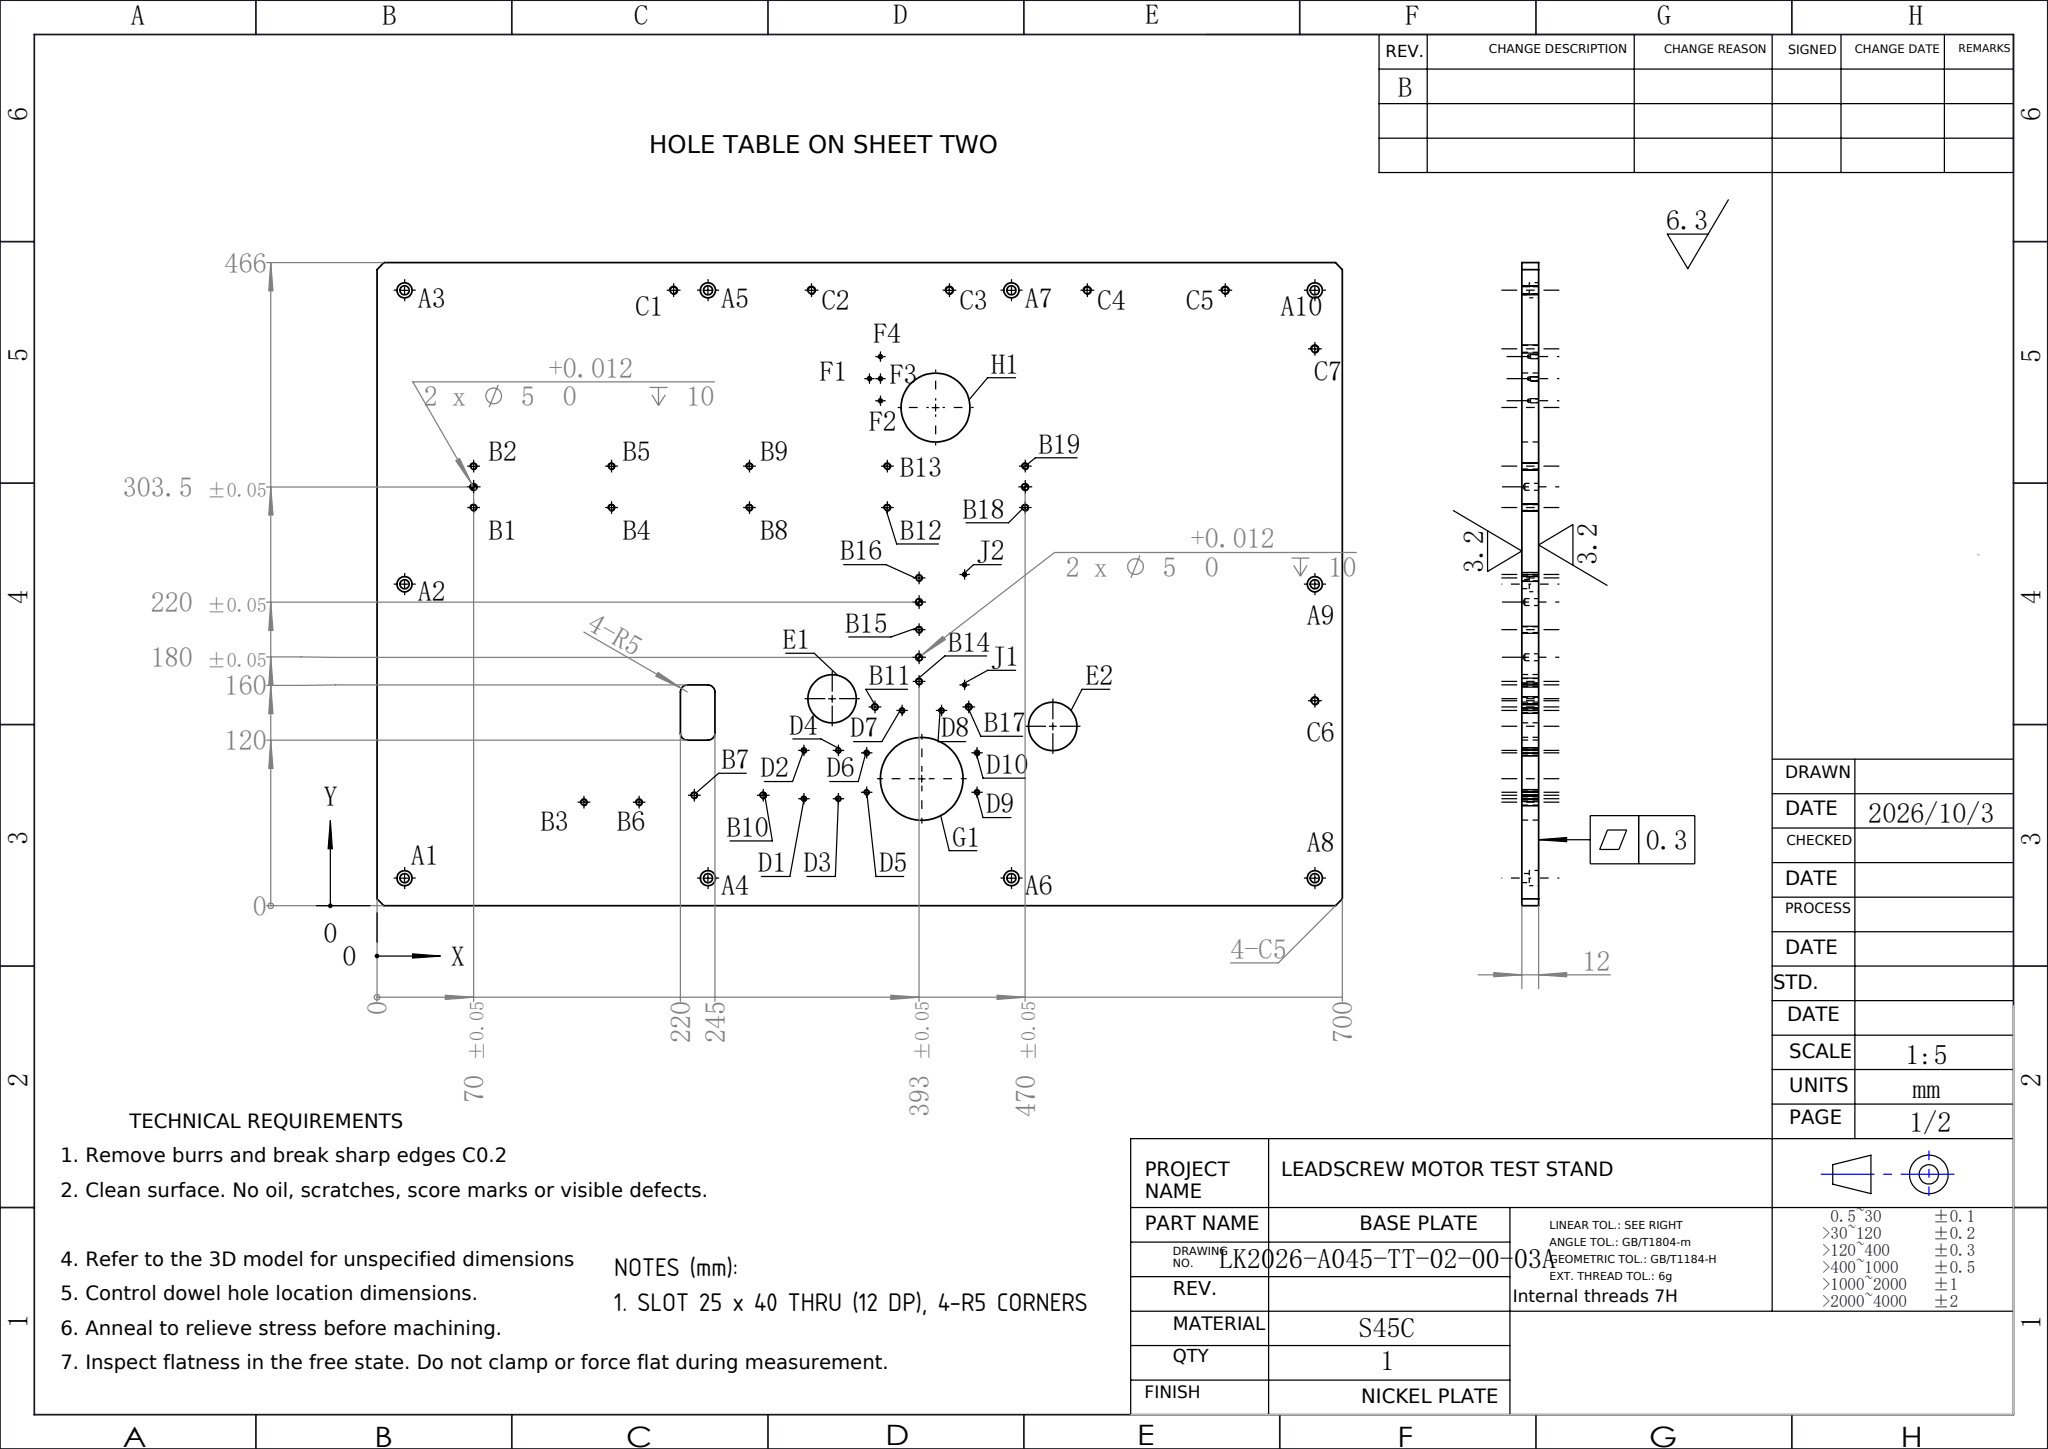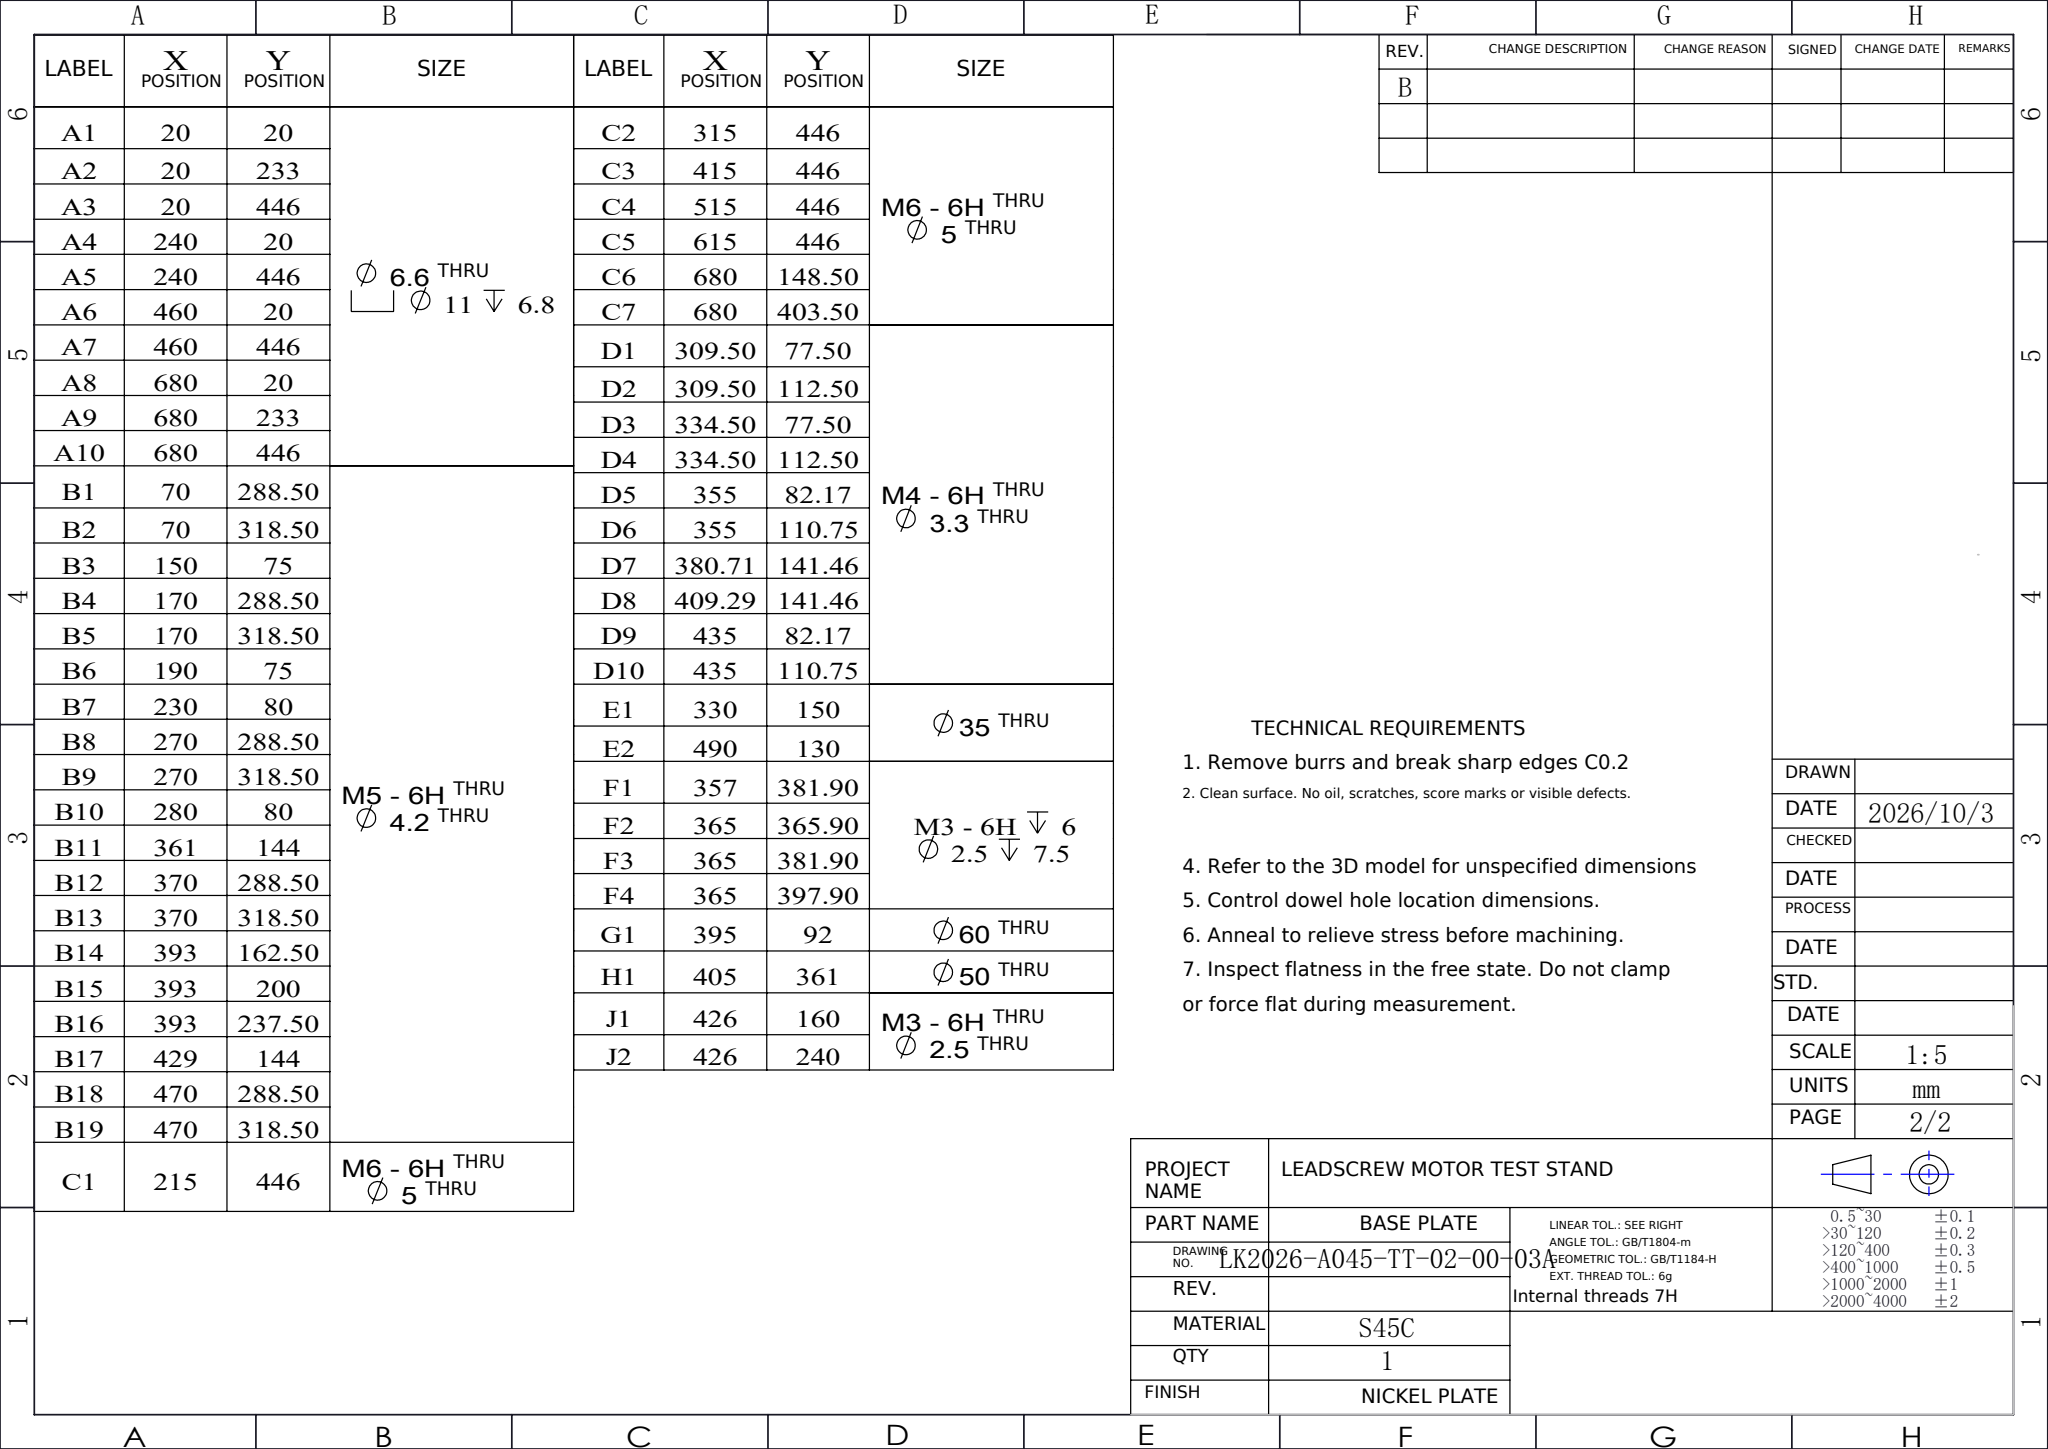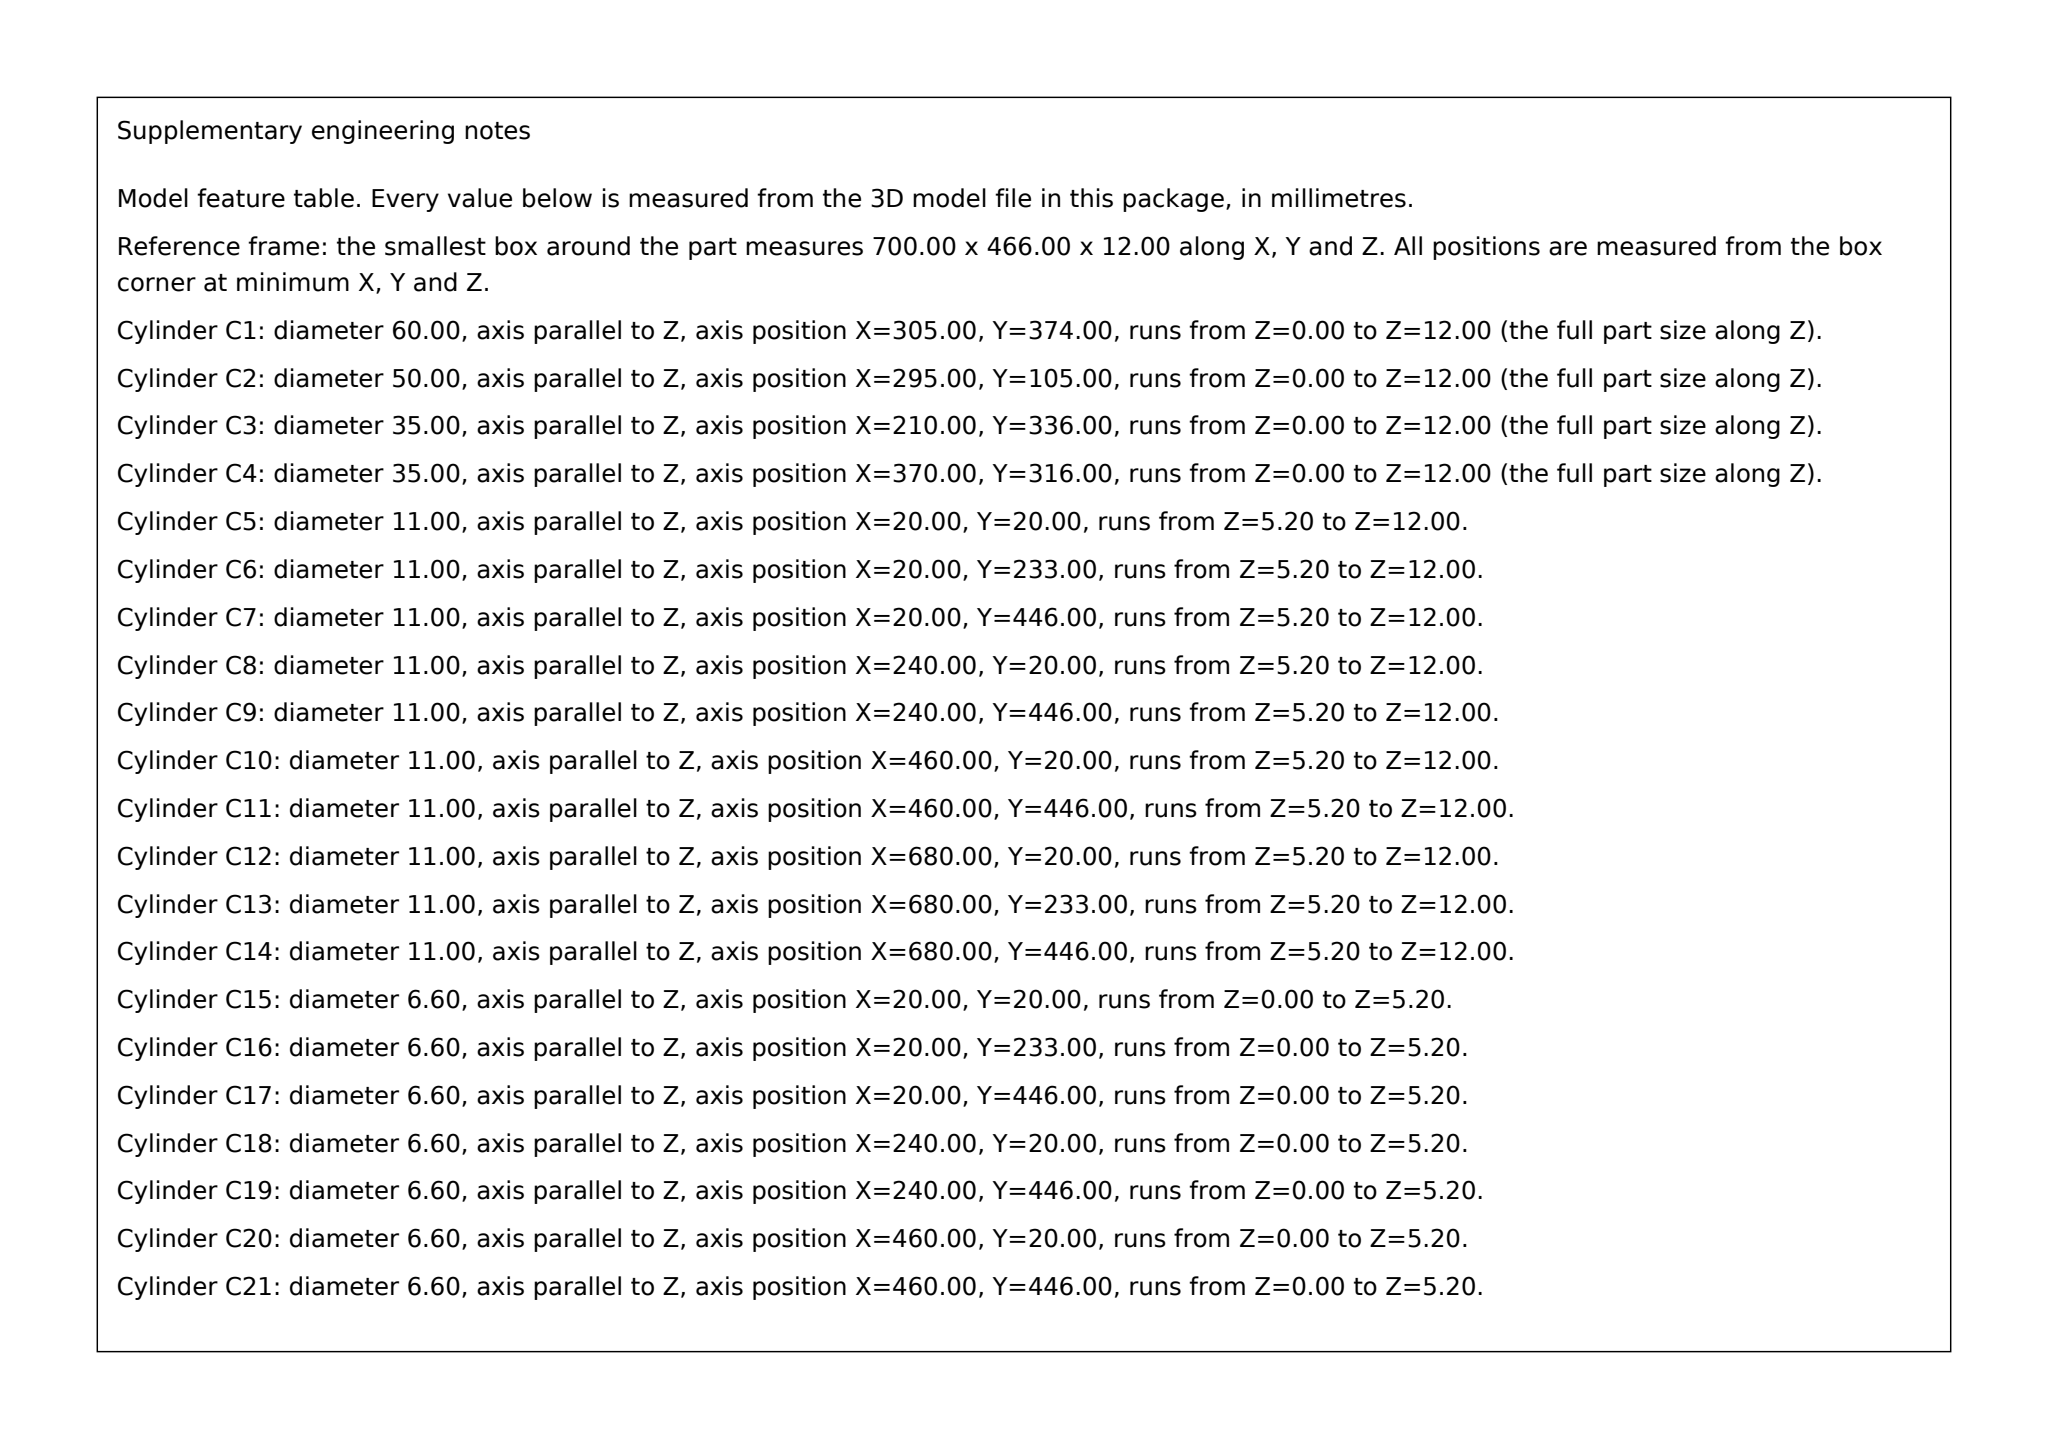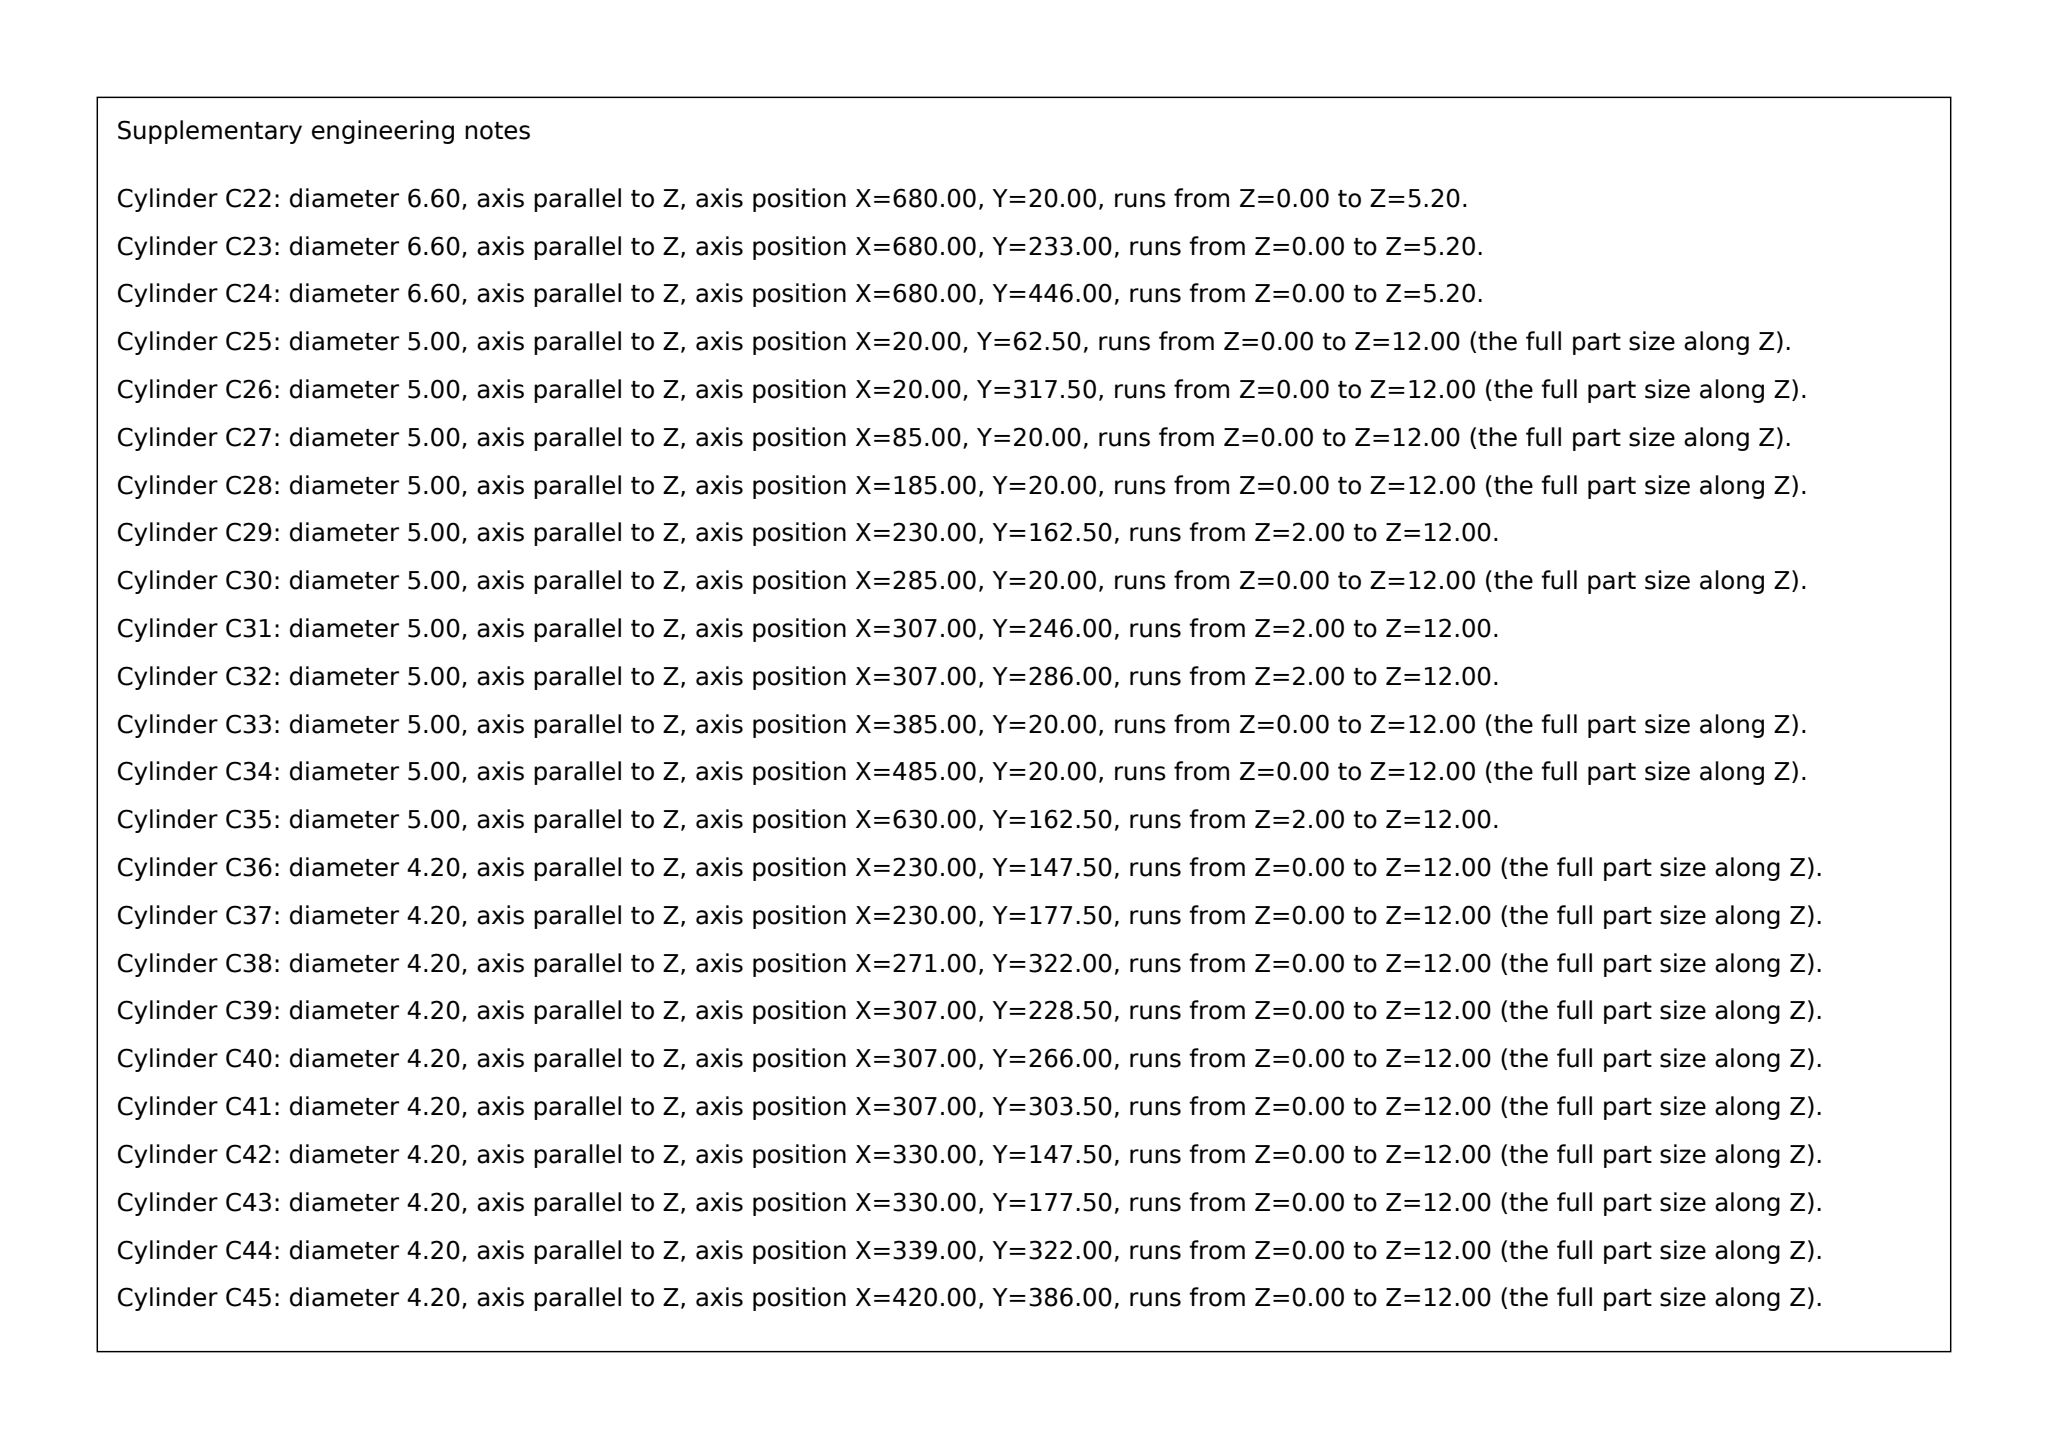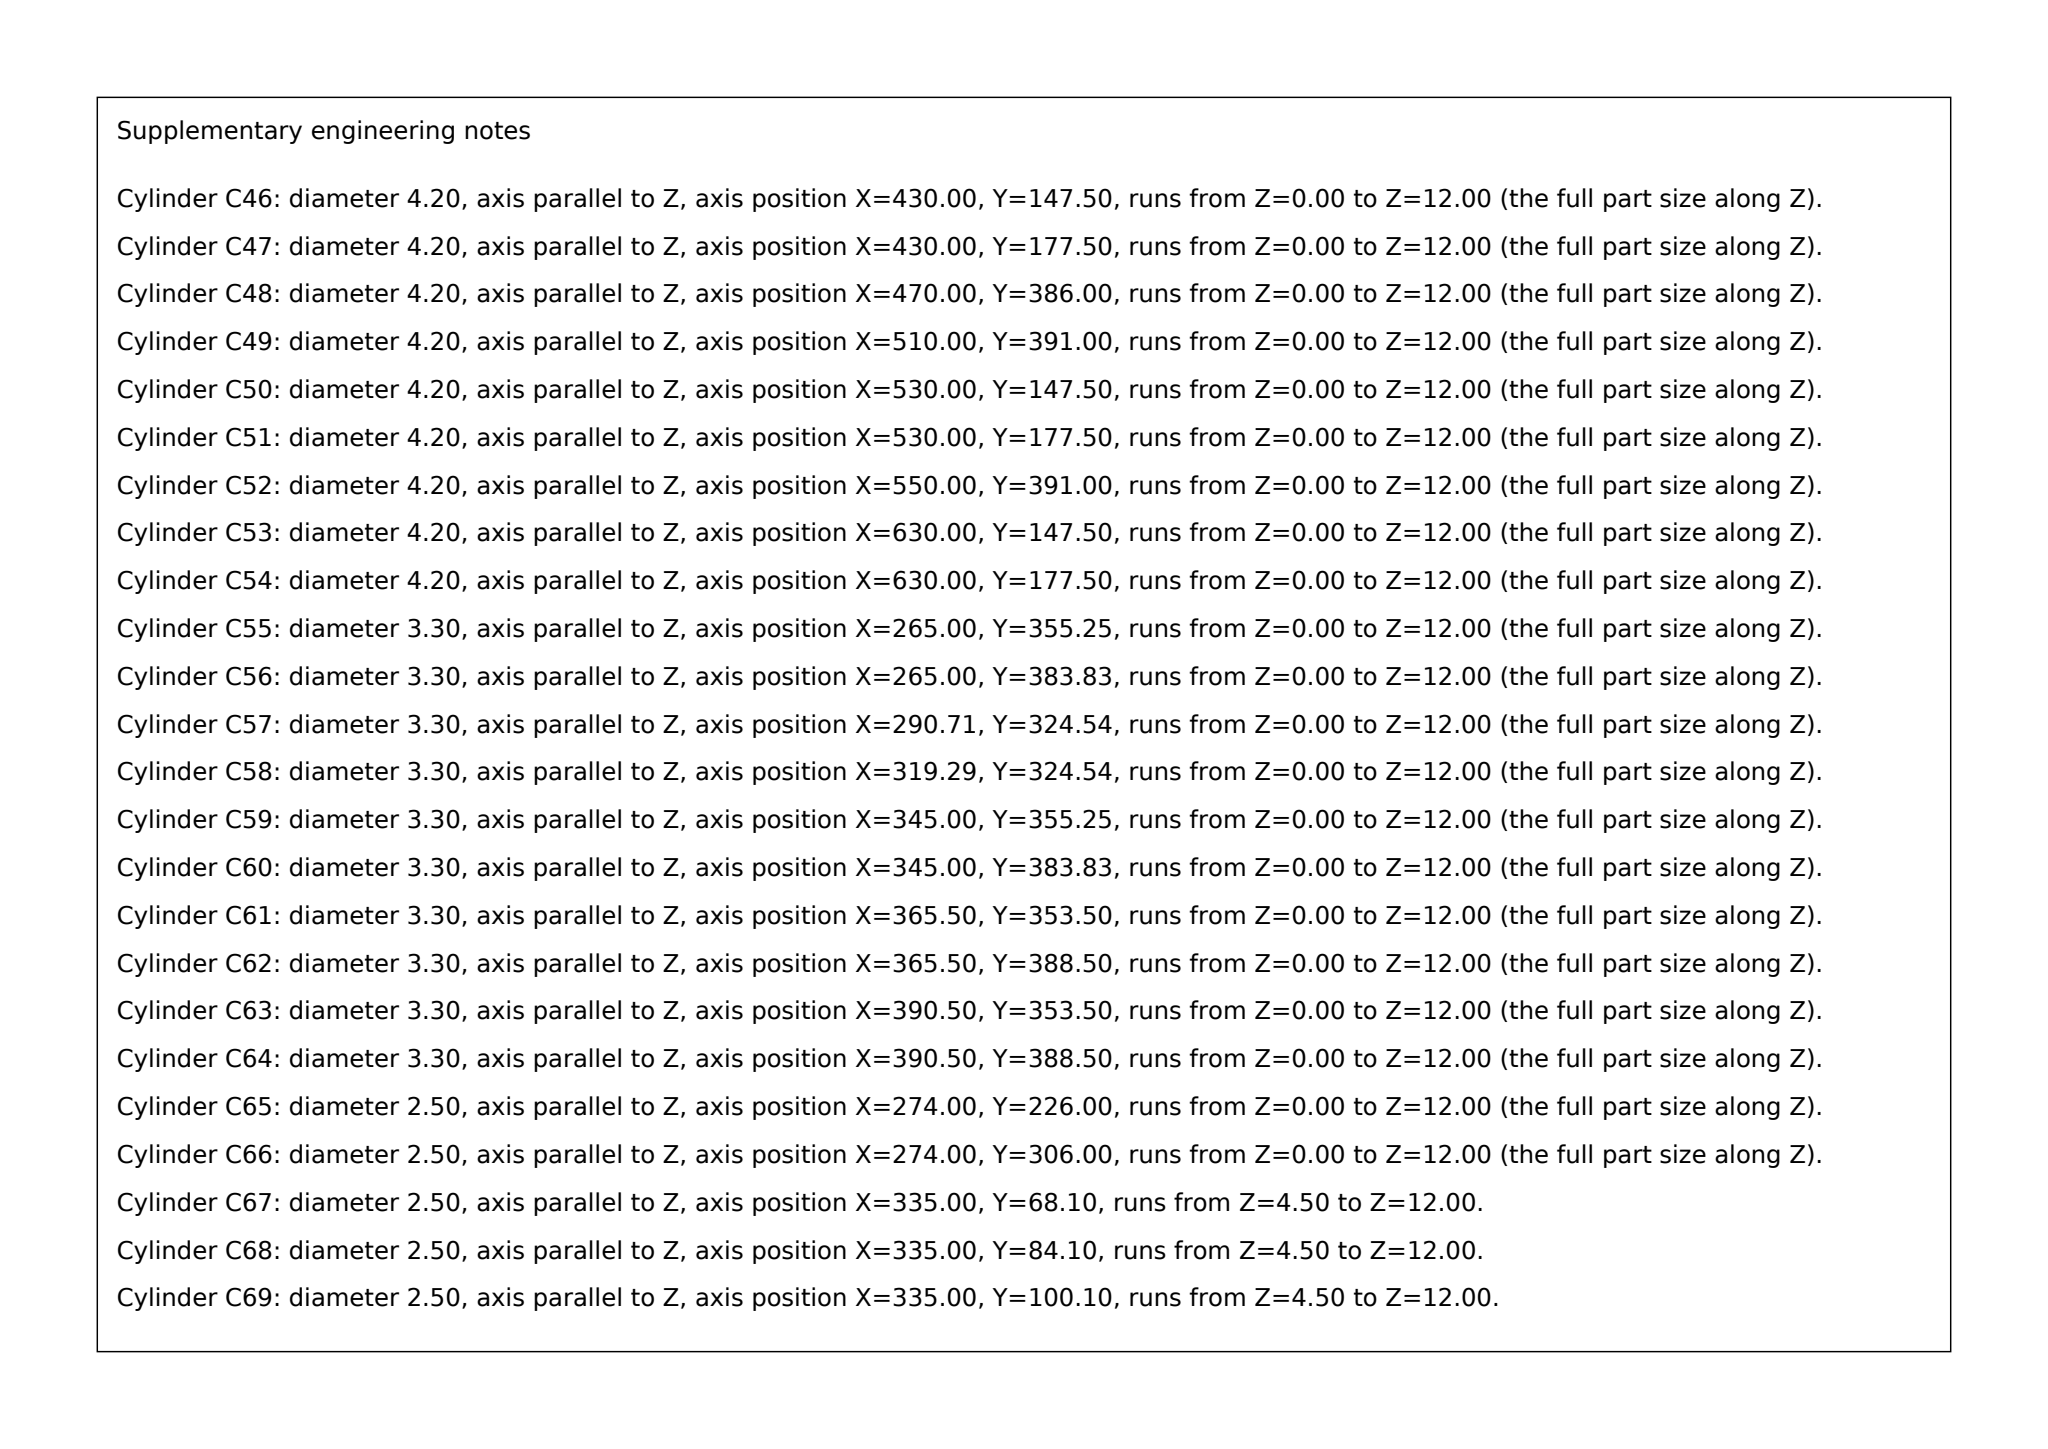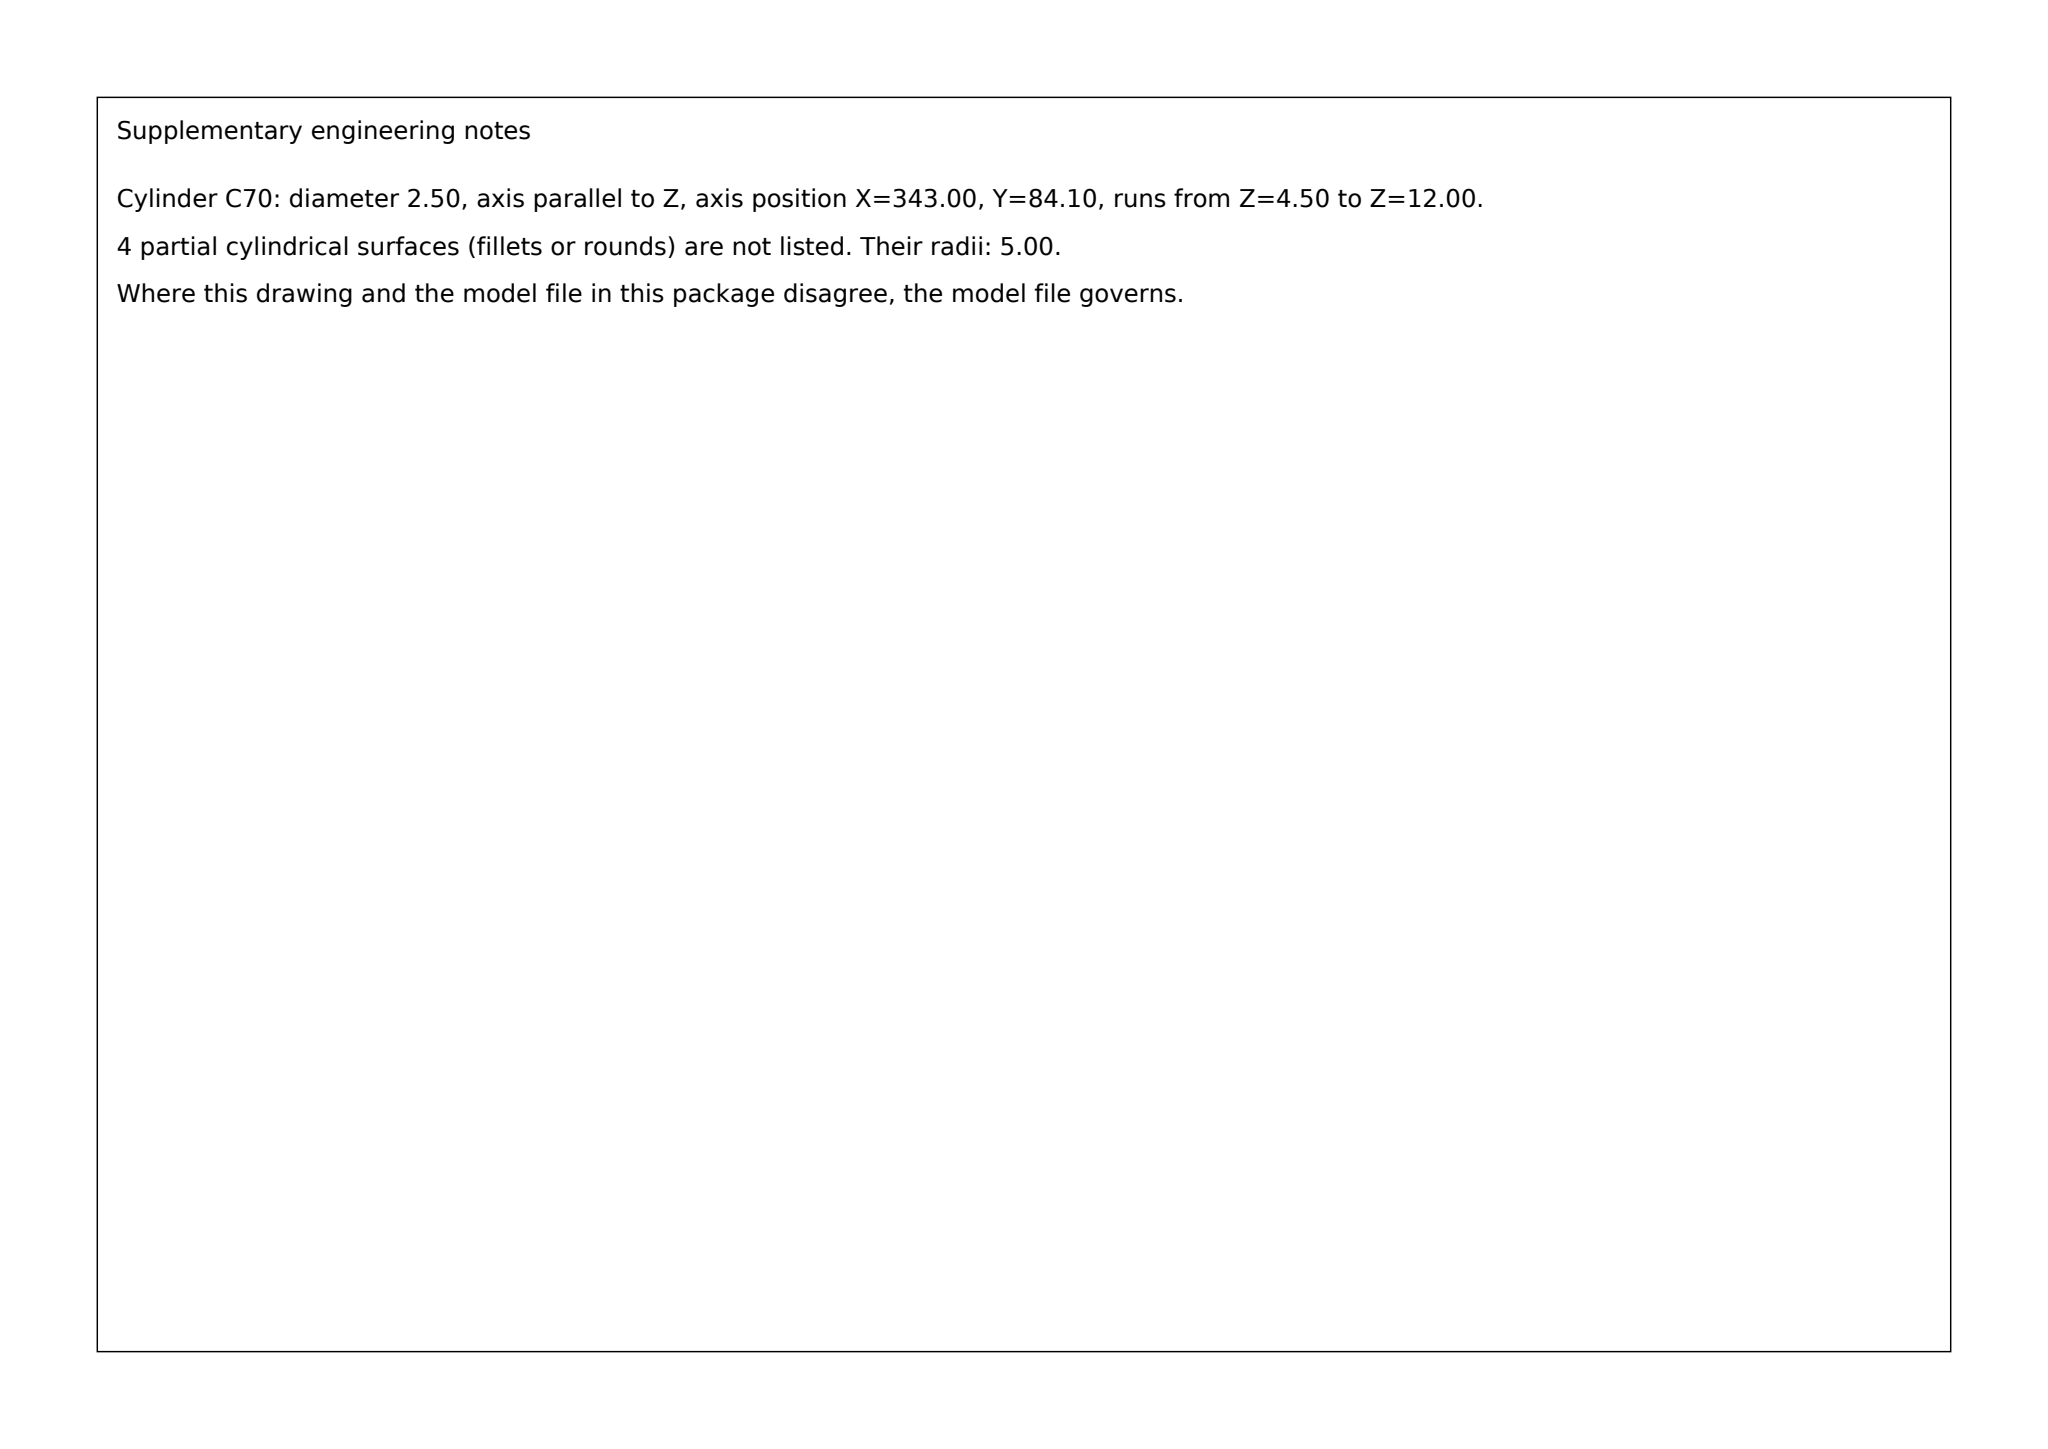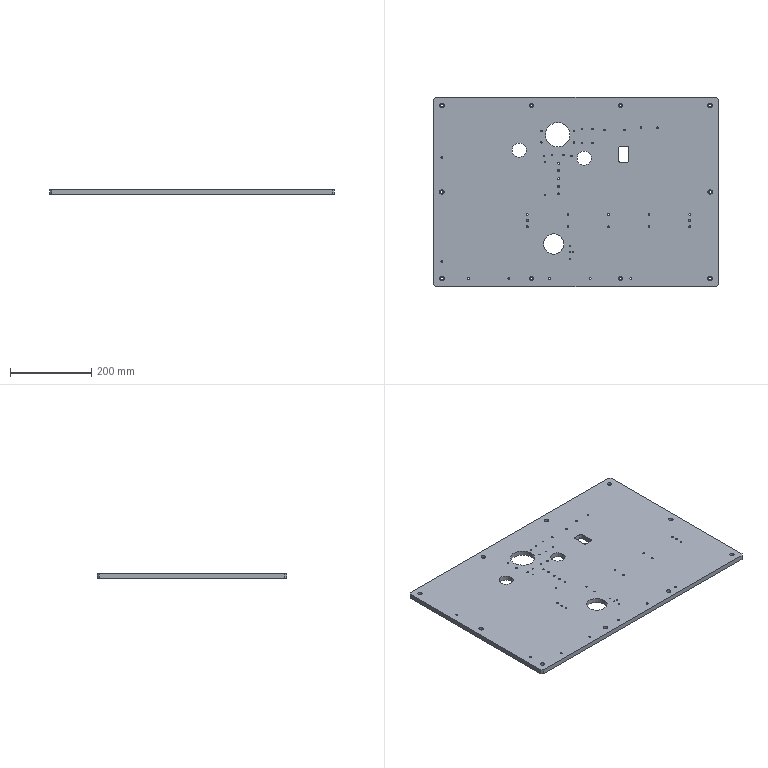Part | SolidWorks | mm | 1 solid | 184 faces | box 700 x 466 x 12 mm | volume 3806305 mm3 | cylinder 144 | plane 24 | cone 16 | commonest cylinder face diameters 4.2 x38 5 x22 3.3 x20 11 x20 6.6 x20 2.5 x12 35 x4 10 x4
Drawing notes:
SLOT 25 x 40 THRU (12 DP), 4-R5 CORNERS | from the solid: Planes x=455/480 and y=306/346 give 25x40 opening; only z planes 0, 5.2 (CBOREs) and 12 exist, so slot is full 12 thk
build123d program:
from build123d import *

# Parameters (mm, degrees)
SKETCH1_W                                       = 700
SKETCH1_H                                       = 466
BOSS_EXTRUDE1_DEPTH                             = 6
SKETCH2_R                                       = 30
CUT_EXTRUDE1_DEPTH                              = 421.634
SKETCH3_W                                       = 25
SKETCH3_H                                       = 40
CUT_EXTRUDE2_DEPTH                              = 421.634
M5_TAPPED_HOLE1_D                               = 4.2
M5_TAPPED_HOLE2_D                               = 4.2
M5_TAPPED_HOLE3_D                               = 4.2
M5_TAPPED_HOLE4_D                               = 4.2
F_5_0_MM_DOWEL_HOLE1_D                          = 5
F_5_0_MM_DOWEL_HOLE1_DEPTH                      = 10
F_5_0_MM_DOWEL_HOLE1_TIP                        = 1.502
M3_TAPPED_HOLE1_D                               = 2.5
M3_TAPPED_HOLE1_DEPTH                           = 7.5
M3_TAPPED_HOLE1_TIP                             = 0.7511
FILLET1_R                                       = 5
SKETCH18_R                                      = 25
SKETCH18_R_2                                    = 17.5
CUT_EXTRUDE3_DEPTH                              = 421.634
F_5_0_MM_DOWEL_HOLE2_D                          = 5
F_5_0_MM_DOWEL_HOLE2_DEPTH                      = 10
F_5_0_MM_DOWEL_HOLE2_TIP                        = 1.502
M5_TAPPED_HOLE5_D                               = 4.2
CHAMFER1_SIZE                                   = 5
M6_HEX_SOCKET_HEAD_CAP_SCREW_CBORE1_D           = 6.6
M6_HEX_SOCKET_HEAD_CAP_SCREW_CBORE1_CBORE_D     = 11
M6_HEX_SOCKET_HEAD_CAP_SCREW_CBORE1_CBORE_DEPTH = 6.8
M4_TAPPED_HOLE1_D                               = 3.3
M6_TAPPED_HOLE1_D                               = 5
M3_TAPPED_HOLE2_D                               = 2.5
M4_TAPPED_HOLE3_D                               = 3.3


with BuildPart() as part:
    # Sketch1 → Boss-Extrude1 (new, symmetric)
    with BuildSketch(Plane.XY):
        Rectangle(SKETCH1_W, SKETCH1_H)
    extrude(amount=BOSS_EXTRUDE1_DEPTH, both=True)

    # Sketch2 → Cut-Extrude1 (cut, through all)
    with BuildSketch(Plane.XY.offset(6)):
        with Locations((-45, 141)):
            Circle(SKETCH2_R)
    extrude(amount=-CUT_EXTRUDE1_DEPTH, mode=Mode.SUBTRACT)

    # Sketch3 → Cut-Extrude2 (cut, through all)
    with BuildSketch(Plane.XY.offset(6)):
        with Locations((117.5, 93)):
            Rectangle(SKETCH3_W, SKETCH3_H)
    extrude(amount=-CUT_EXTRUDE2_DEPTH, mode=Mode.SUBTRACT)

    # M5 Tapped Hole1 (through all)
    with Locations(Plane.XY.offset(6)):
        with Locations((160, 158), (200, 158)):
            Hole(M5_TAPPED_HOLE1_D / 2)

    # M5 Tapped Hole2 (through all)
    with Locations(Plane.XY.offset(6)):
        with Locations((70, 153), (120, 153)):
            Hole(M5_TAPPED_HOLE2_D / 2)

    # M5 Tapped Hole3 (through all)
    with Locations(Plane.XY.offset(6)):
        with Locations((-79, 89), (-11, 89)):
            Hole(M5_TAPPED_HOLE3_D / 2)

    # M5 Tapped Hole4 (through all)
    with Locations(Plane.XY.offset(6)):
        with Locations((280, -85.5), (180, -85.5), (80, -85.5), (-20, -85.5), (-120, -85.5), (-20, -55.5), (80, -55.5), (180, -55.5), (280, -55.5), (-120, -55.5)):
            Hole(M5_TAPPED_HOLE4_D / 2)

    # 5.0 mm Dowel Hole1
    with Locations(Plane.XY.offset(6)):
        with Locations((280, -70.5), (-120, -70.5)):
            Hole(F_5_0_MM_DOWEL_HOLE1_D / 2, depth=F_5_0_MM_DOWEL_HOLE1_DEPTH)
            with Locations((0, 0, -(F_5_0_MM_DOWEL_HOLE1_DEPTH + F_5_0_MM_DOWEL_HOLE1_TIP / 2))):  # 118° drill point
                Cone(0, F_5_0_MM_DOWEL_HOLE1_D / 2, F_5_0_MM_DOWEL_HOLE1_TIP, mode=Mode.SUBTRACT)

    # M3 Tapped Hole1
    with Locations(Plane.XY.offset(6)):
        with Locations((-15, -132.9), (-15, -148.9), (-7, -148.9), (-15, -164.9)):
            Hole(M3_TAPPED_HOLE1_D / 2, depth=M3_TAPPED_HOLE1_DEPTH)
            with Locations((0, 0, -(M3_TAPPED_HOLE1_DEPTH + M3_TAPPED_HOLE1_TIP / 2))):  # 118° drill point
                Cone(0, M3_TAPPED_HOLE1_D / 2, M3_TAPPED_HOLE1_TIP, mode=Mode.SUBTRACT)

    # Fillet1
    fillet1_edges = [part.edges().sort_by_distance(p)[0] for p in [
        (130, 113, 0),
        (130, 73, 0),
        (105, 73, 0),
        (105, 113, 0),
    ]]
    fillet(fillet1_edges, radius=FILLET1_R)

    # Sketch18 → Cut-Extrude3 (cut, through all)
    with BuildSketch(Plane.XY.offset(6)):
        with Locations((-55, -128)):
            Circle(SKETCH18_R)
        with Locations((20, 83)):
            Circle(SKETCH18_R_2)
        with Locations((-140, 103)):
            Circle(SKETCH18_R_2)
    extrude(amount=-CUT_EXTRUDE3_DEPTH, mode=Mode.SUBTRACT)

    # 5.0 mm Dowel Hole2
    with Locations(Plane.XY.offset(6)):
        with Locations((-43, 13), (-43, 53)):
            Hole(F_5_0_MM_DOWEL_HOLE2_D / 2, depth=F_5_0_MM_DOWEL_HOLE2_DEPTH)
            with Locations((0, 0, -(F_5_0_MM_DOWEL_HOLE2_DEPTH + F_5_0_MM_DOWEL_HOLE2_TIP / 2))):  # 118° drill point
                Cone(0, F_5_0_MM_DOWEL_HOLE2_D / 2, F_5_0_MM_DOWEL_HOLE2_TIP, mode=Mode.SUBTRACT)

    # M5 Tapped Hole5 (through all)
    with Locations(Plane.XY.offset(6)):
        with Locations((-43, -4.5), (-43, 70.5), (-43, 33)):
            Hole(M5_TAPPED_HOLE5_D / 2)

    # Chamfer1
    chamfer1_edges = [part.edges().sort_by_distance(p)[0] for p in [
        (350, -233, 0),
        (-350, -233, 0),
        (-350, 233, 0),
        (350, 233, 0),
    ]]
    chamfer(chamfer1_edges, length=CHAMFER1_SIZE)

    # M6 Hex Socket Head Cap Screw CBORE1 (through all)
    with Locations(Plane.XY.offset(6)):
        with Locations((-330, 213), (330, -213), (-330, -213), (330, 213), (-330, 0), (330, 0), (-110, 213), (110, 213), (-110, -213), (110, -213)):
            CounterBoreHole(M6_HEX_SOCKET_HEAD_CAP_SCREW_CBORE1_D / 2, M6_HEX_SOCKET_HEAD_CAP_SCREW_CBORE1_CBORE_D / 2, M6_HEX_SOCKET_HEAD_CAP_SCREW_CBORE1_CBORE_DEPTH)

    # M4 Tapped Hole1 (through all)
    with Locations(Plane.XY.offset(6)):
        with Locations((15.5, 155.5), (15.5, 120.5), (40.5, 120.5), (40.5, 155.5)):
            Hole(M4_TAPPED_HOLE1_D / 2)

    # M6 Tapped Hole1 (through all)
    with Locations(Plane.XY.offset(6)):
        with Locations((135, -213), (35, -213), (-65, -213), (-165, -213), (-265, -213), (-330, -170.5), (-330, 84.5)):
            Hole(M6_TAPPED_HOLE1_D / 2)

    # M3 Tapped Hole2 (through all)
    with Locations(Plane.XY.offset(6)):
        with Locations((-76, -7), (-76, 73)):
            Hole(M3_TAPPED_HOLE2_D / 2)

    # M4 Tapped Hole3 (through all)
    with Locations(Plane.XY.offset(6)):
        with Locations((-85, 150.834), (-59.293, 91.541), (-30.707, 91.541), (-85, 122.248), (-5, 122.248), (-5, 150.834)):
            Hole(M4_TAPPED_HOLE3_D / 2)


solid = part.part